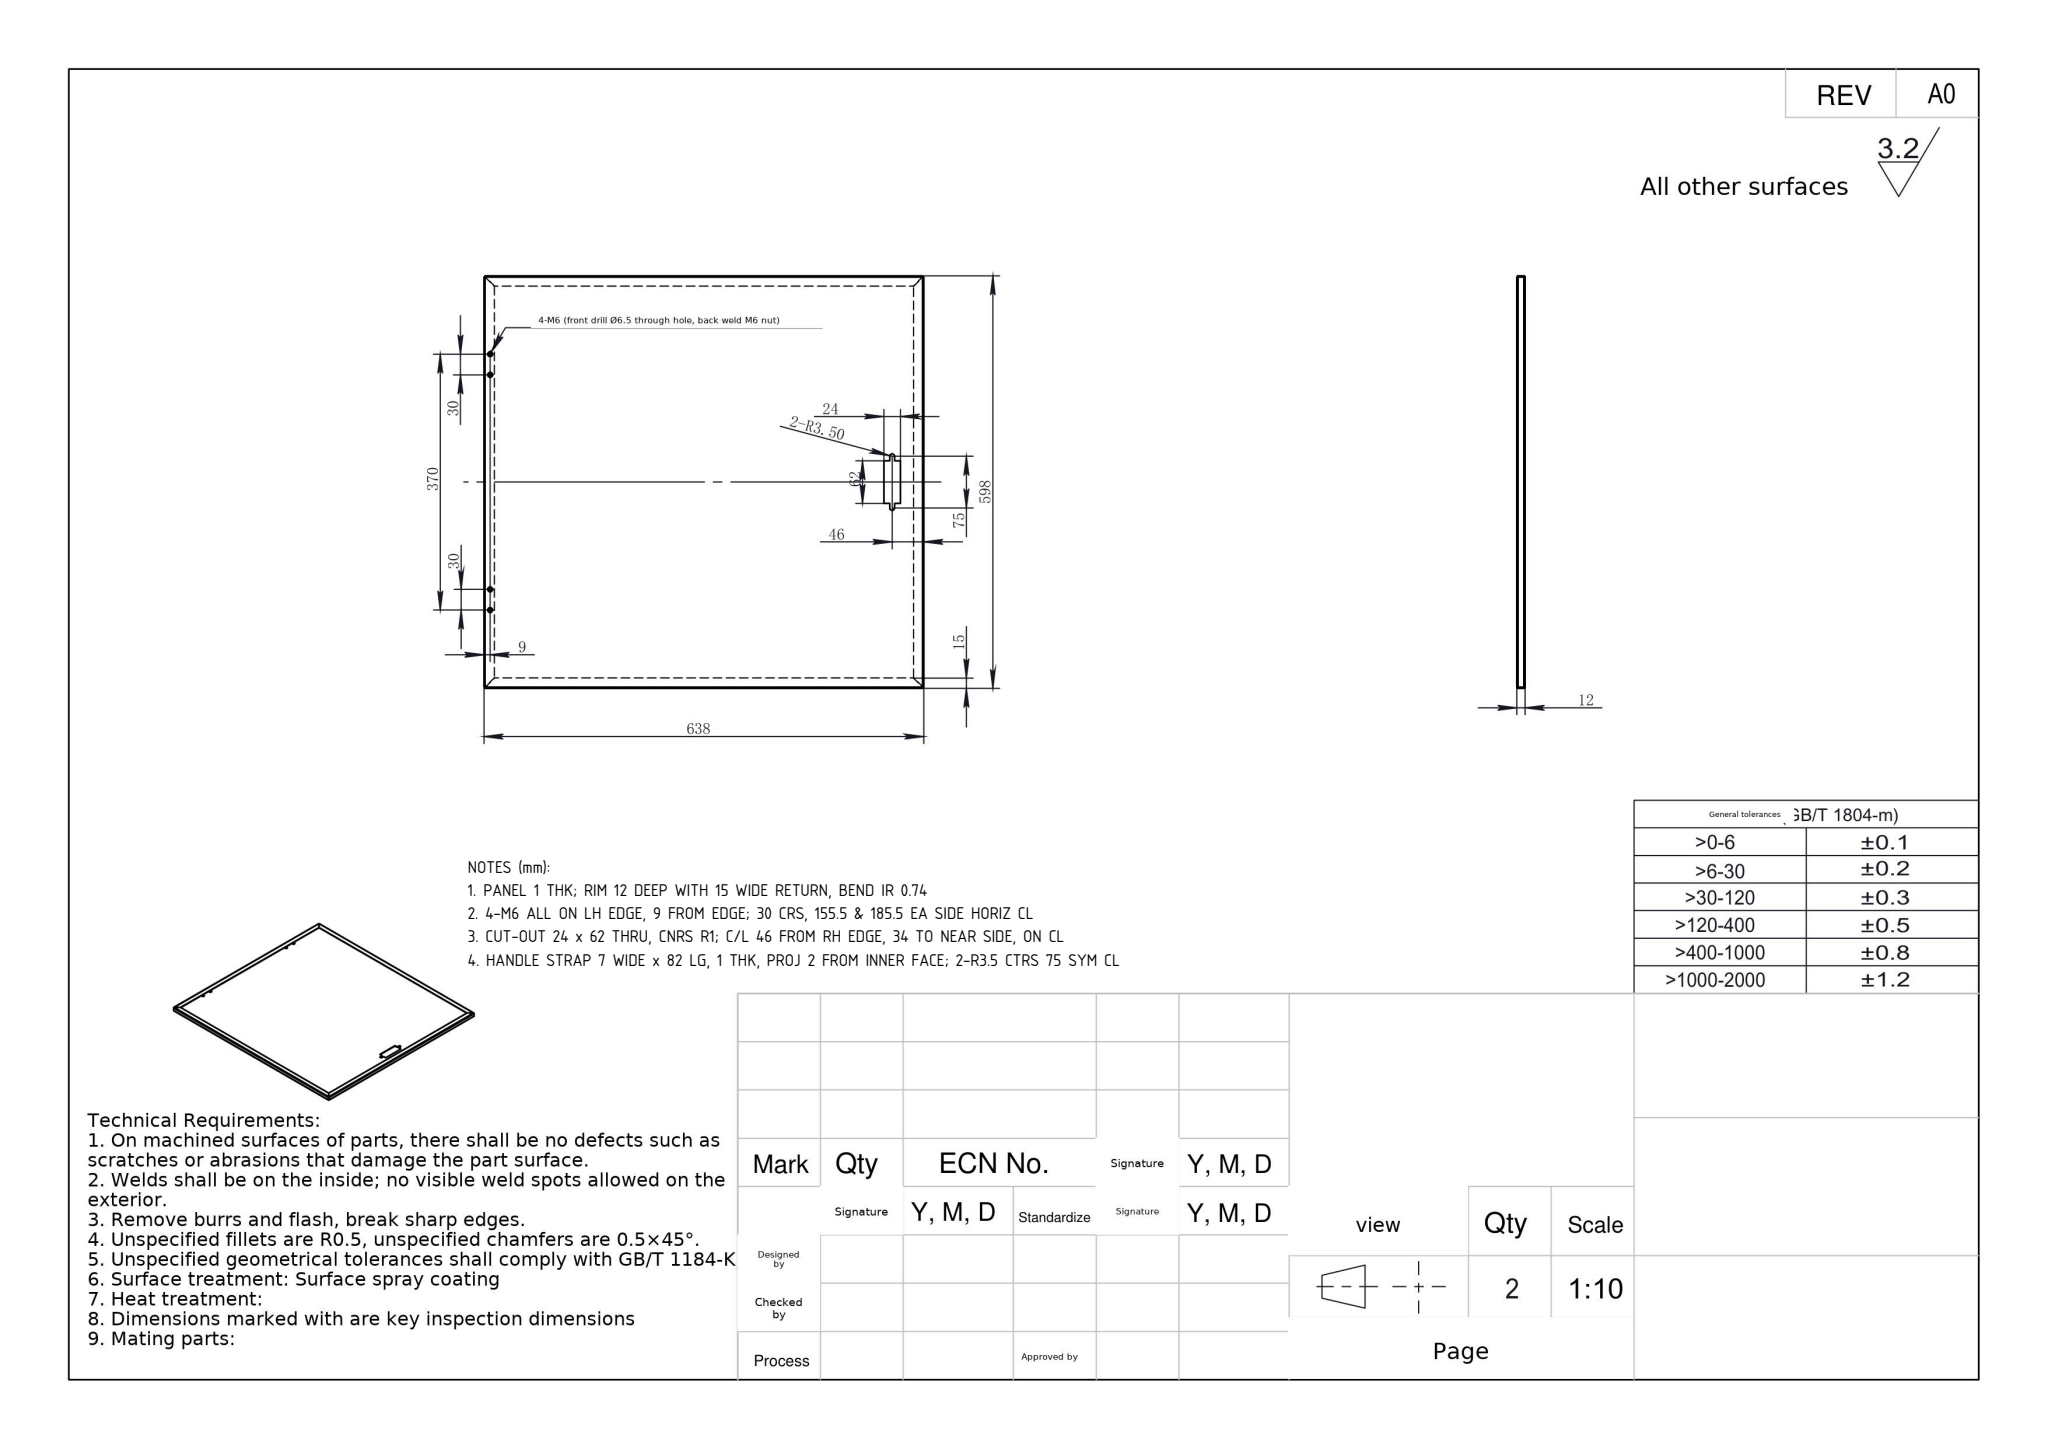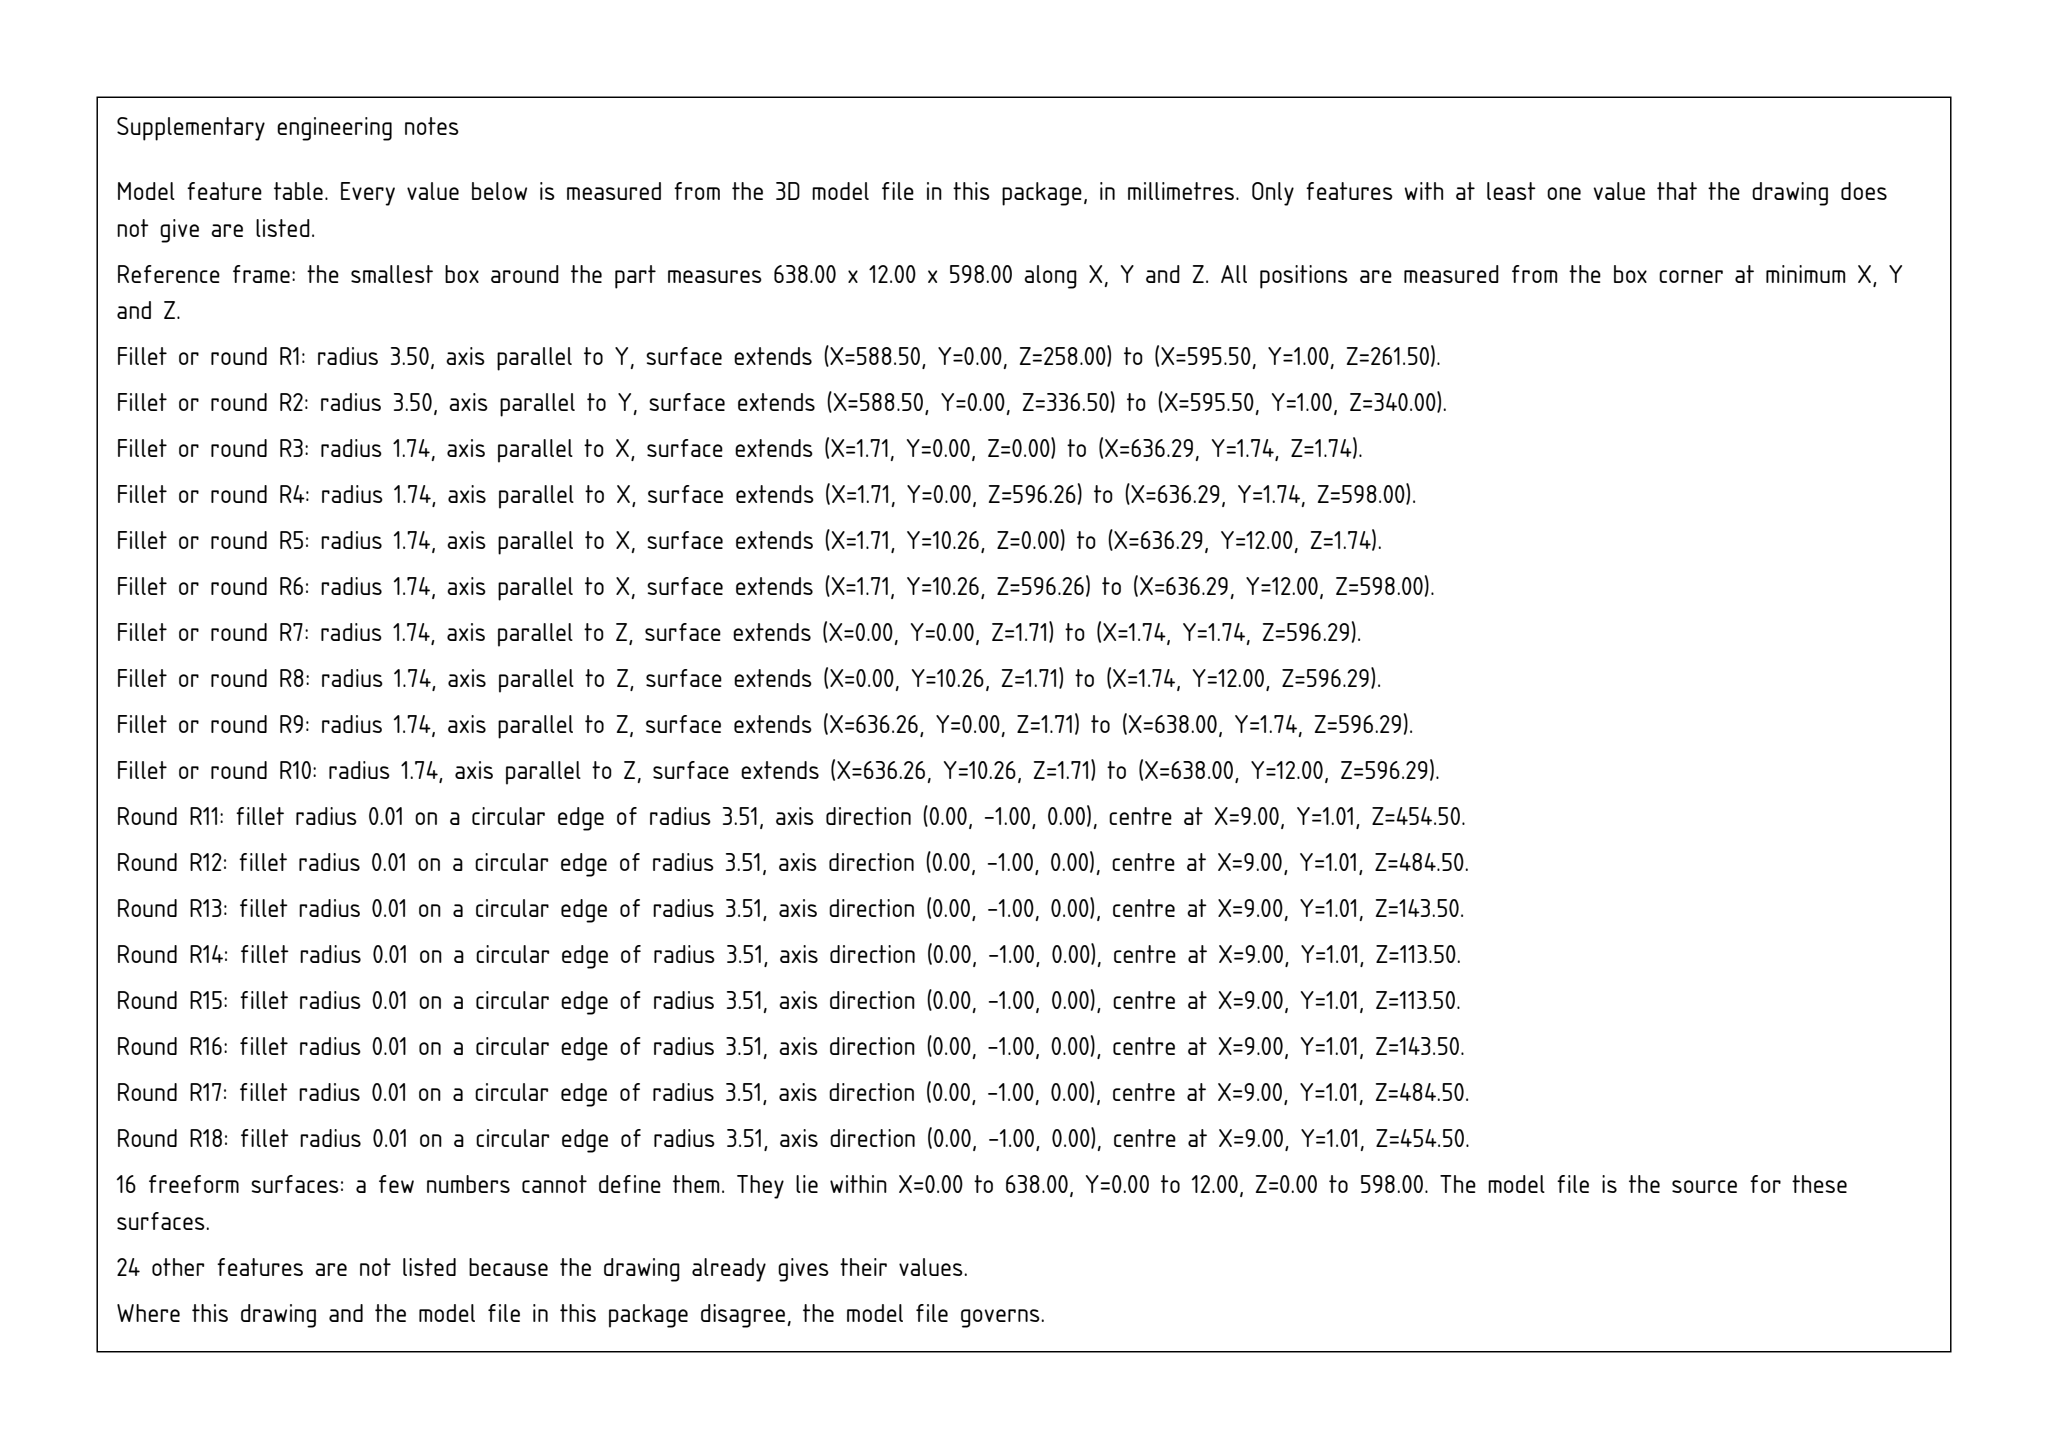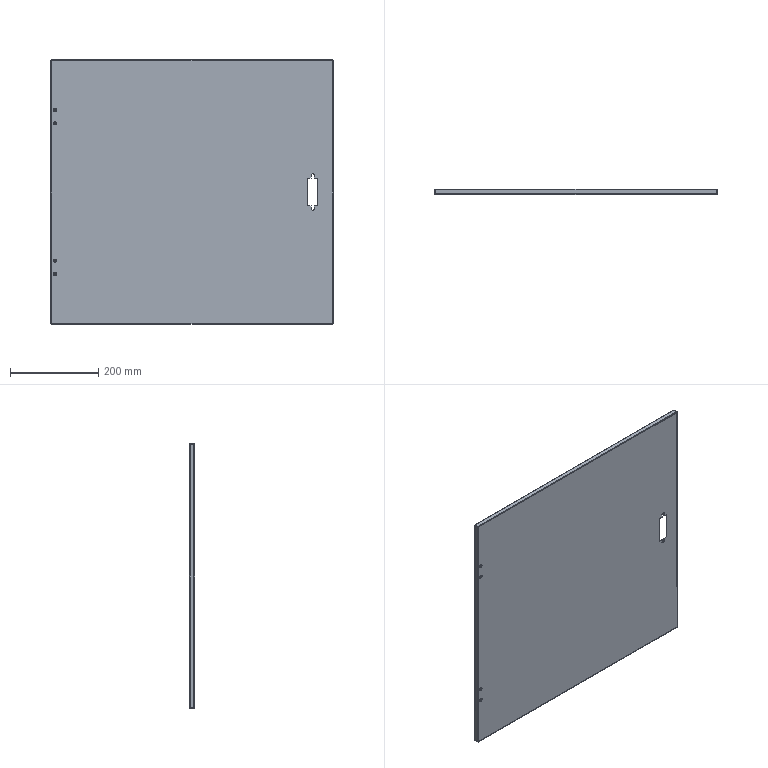Part | SolidWorks | mm | 1 solid | 119 faces | box 638 x 12 x 598 mm | volume 438054 mm3 | plane 52 | cylinder 35 | torus 16 | spline 16 | commonest cylinder face diameters 7 x11 5 x8 3.473 x8 1.473 x8
Drawing notes:
PANEL 1 THK; RIM 12 DEEP WITH 15 WIDE RETURN, BEND IR 0.74 | from the solid: y planes 0.01/1.01 = 1 thk; bbox y 12.02; return flange y 11.01/12.01 to x=15.01 & z=15.01; bend cyls Ø1.473 IR0.74 / Ø3.473 OR1.74
4-M6 ALL ON LH EDGE, 9 FROM EDGE; 30 CRS, 155.5 & 185.5 EA SIDE HORIZ CL | from the solid: Ø5/Ø7 y-axis holes all at x=9.01; z=113.51,143.51,454.51,484.51 (30 within pairs, 371 overall, sym abt CL z=299.01); no holes at RH side
CUT-OUT 24 x 62 THRU, CNRS R1; C/L 46 FROM RH EDGE, 34 TO NEAR SIDE, ON CL | from the solid: x planes 580.01/604.01 (24 wide, C/L 592.01 = 638.02-46, near side 638.02-604.01=34); z planes 268.01/330.01 (62, sym abt 299.01); fillet_radii 1.01 x8
HANDLE STRAP 7 WIDE x 82 LG, 1 THK, PROJ 2 FROM INNER FACE; 2-R3.5 CTRS 75 SYM CL | from the solid: Ø7 cyls axis y at x=592.01, z=261.51 & 336.51, length 1.0; tangent x planes 588.51/595.51 = 7 wide; OAL 82; y planes 1.01 to 3.01